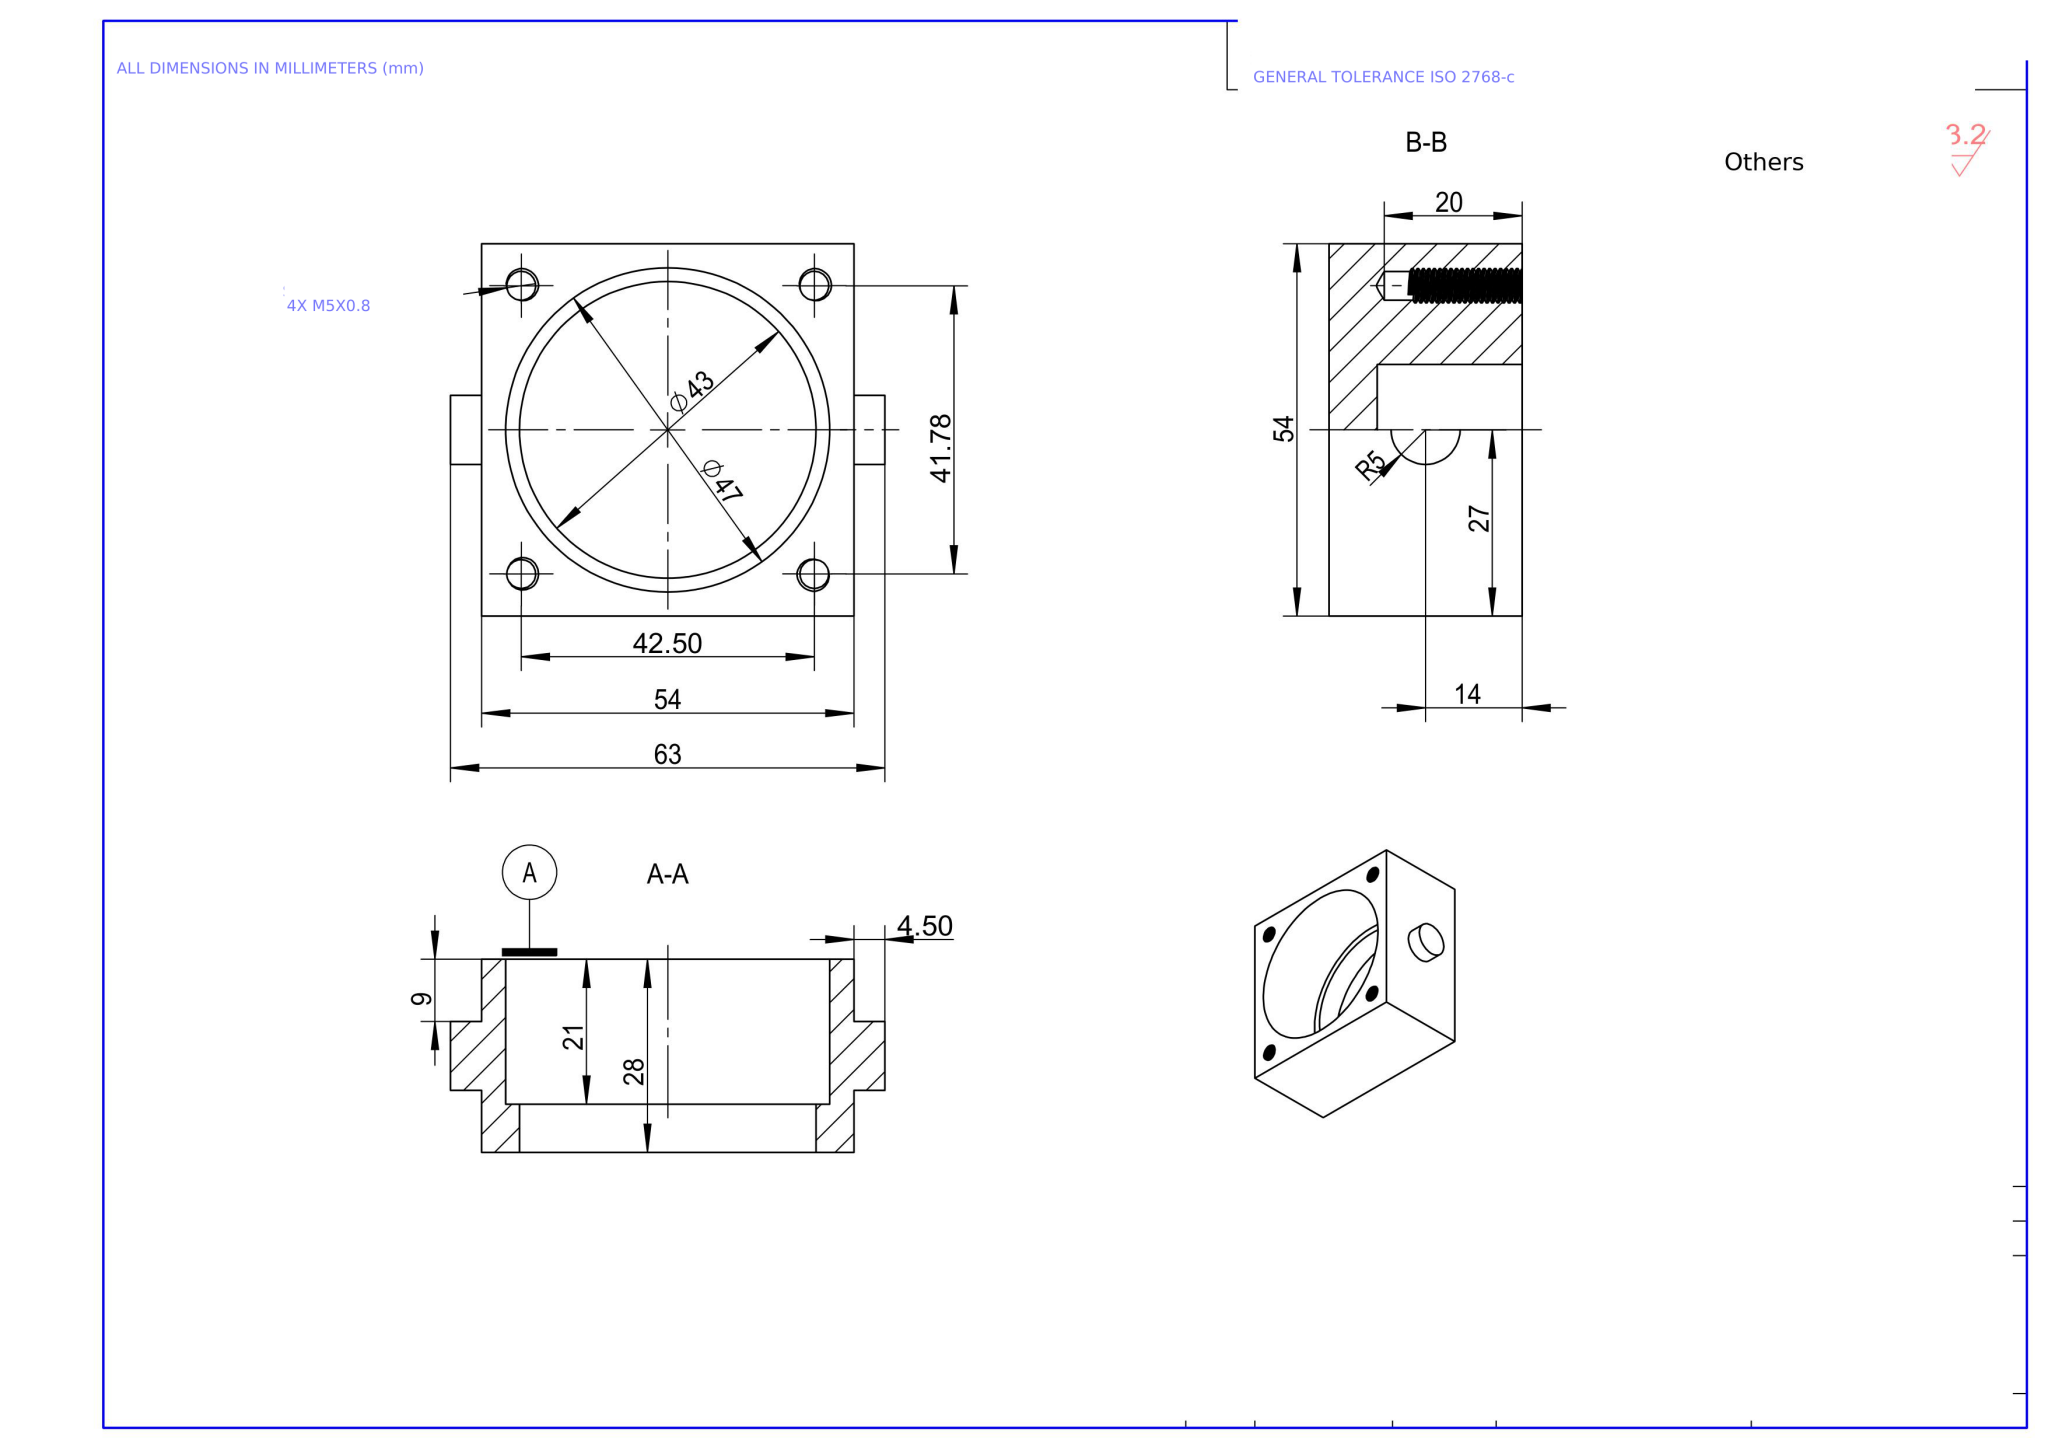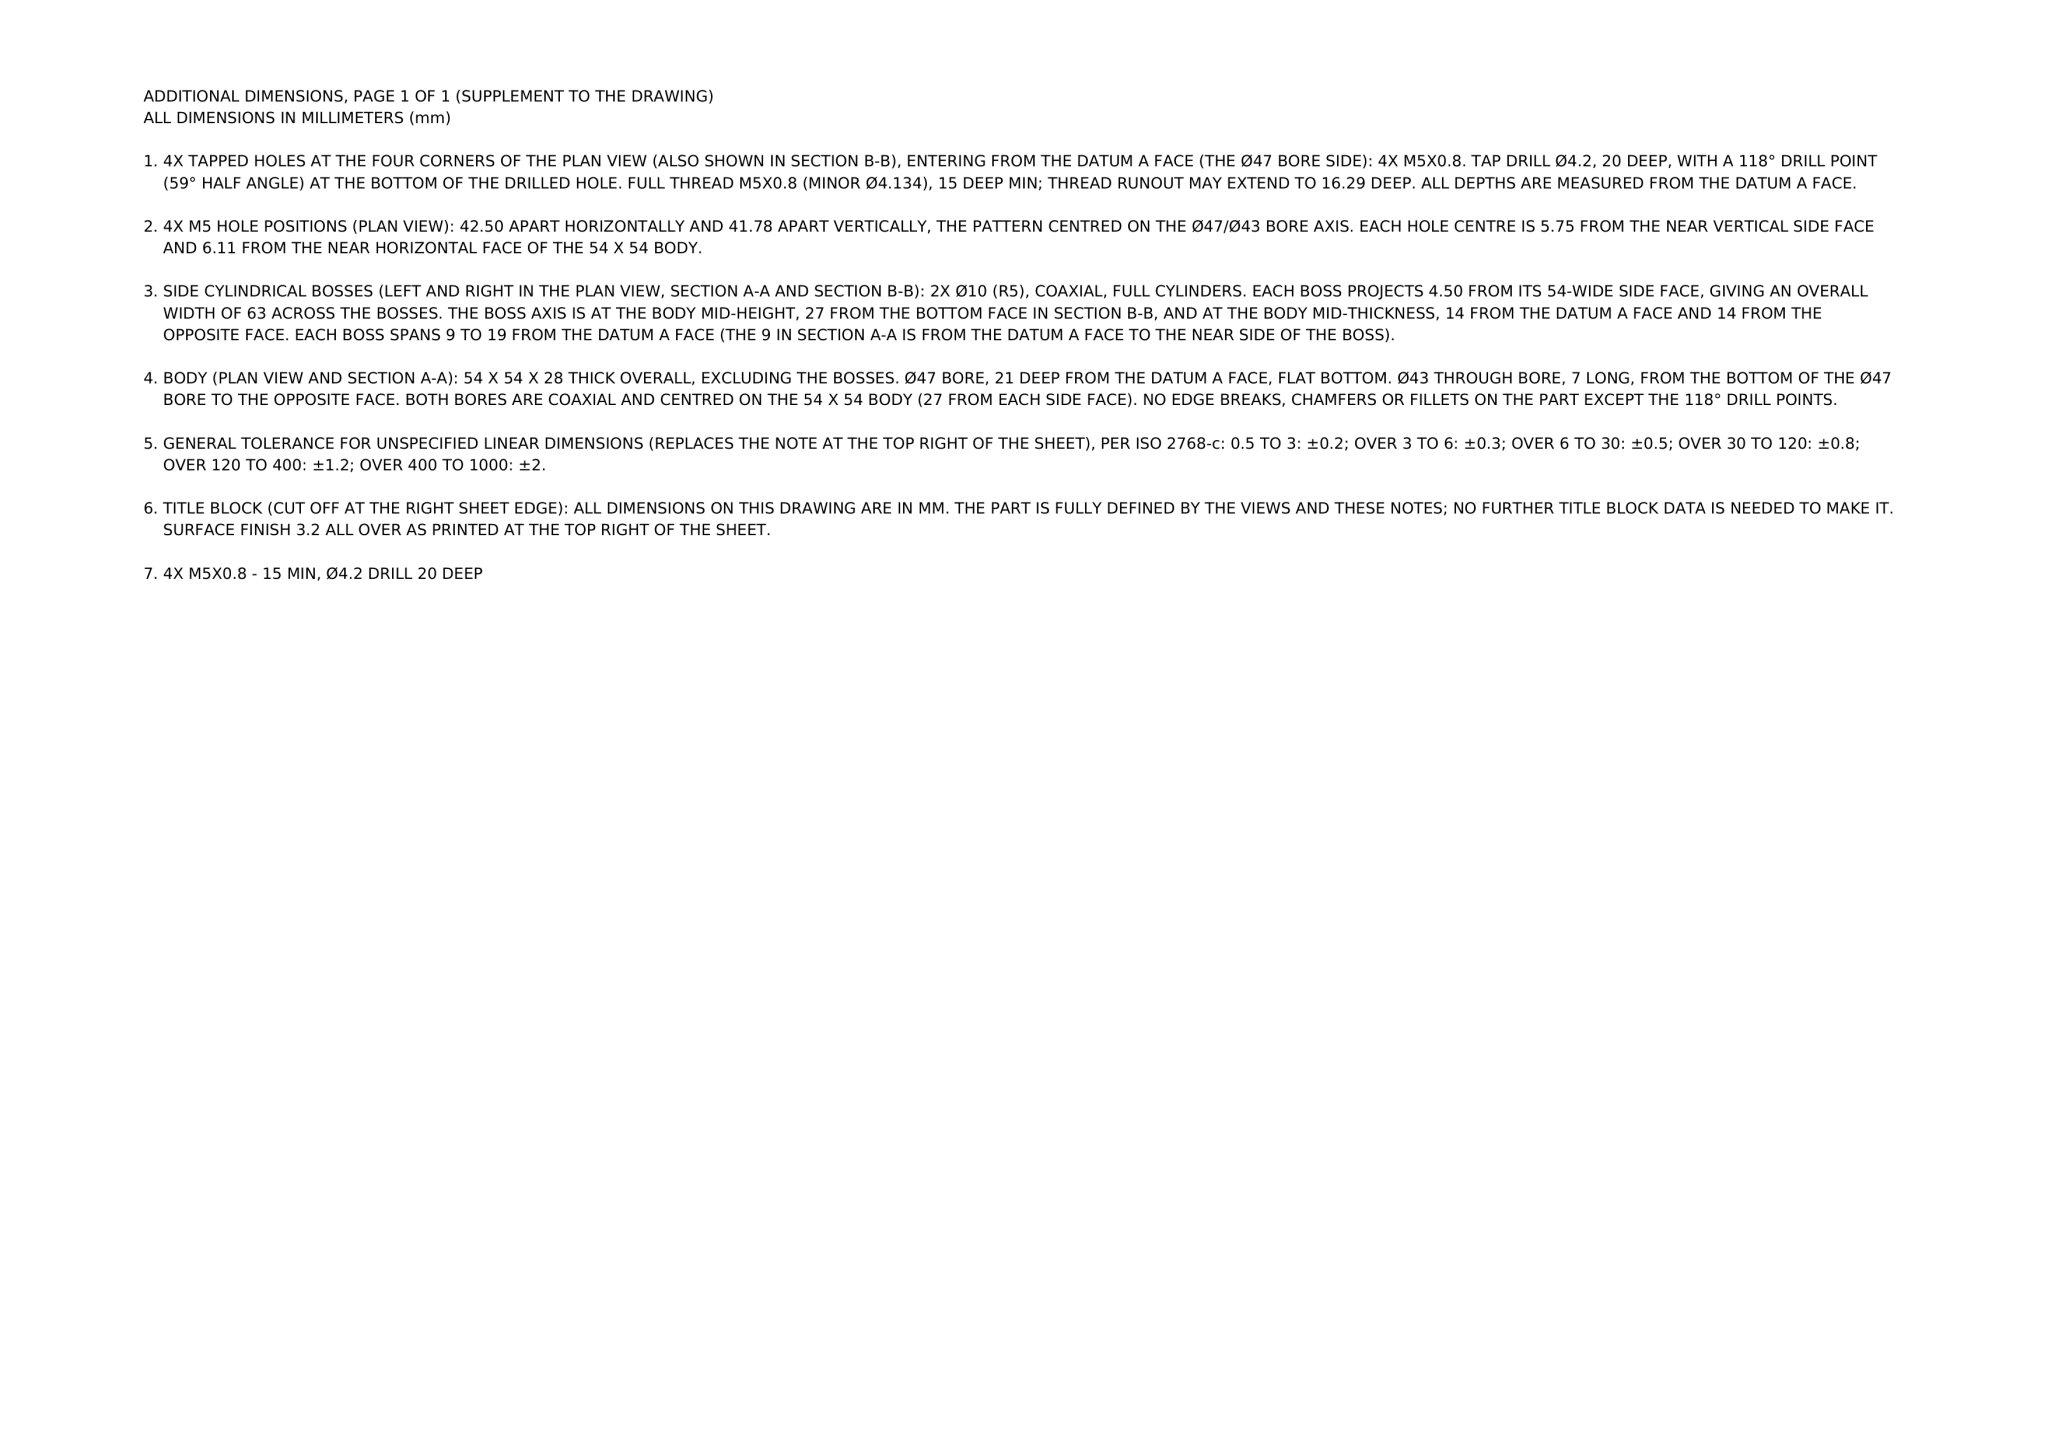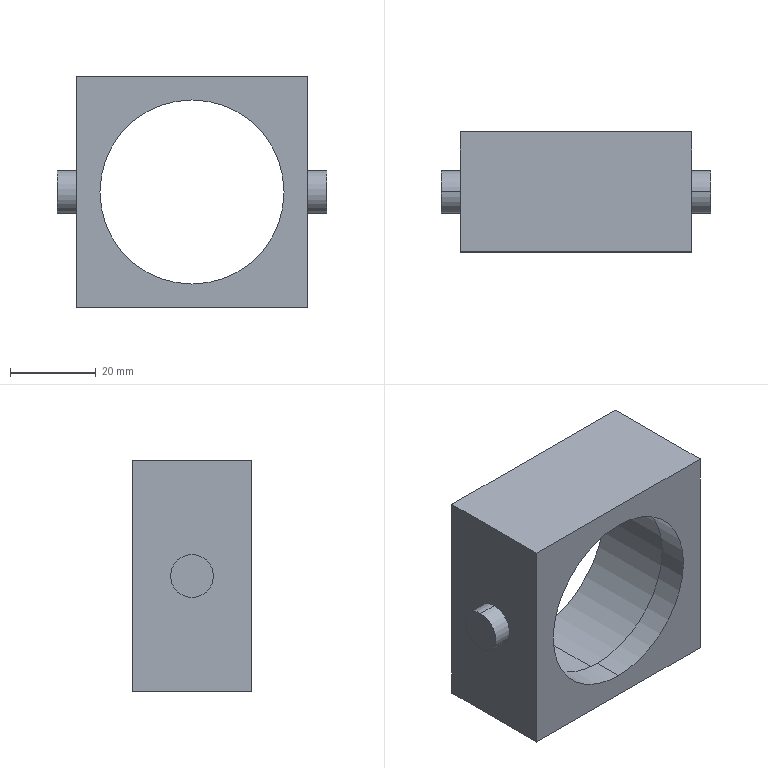Part | NX | mm | 1 solid | 368 faces | box 63 x 28 x 54 mm | volume 34591 mm3 | cylinder 339 | plane 13 | cone 8 | spline 8 | commonest cylinder face diameters 5 x167 4.2 x164 10 x4 47 x2 43 x2